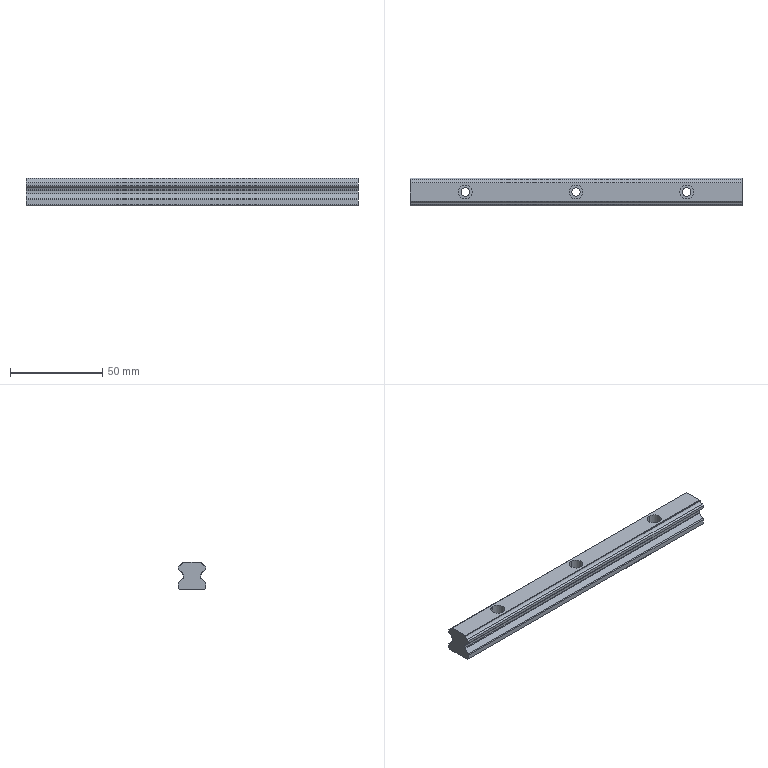Component | SolidWorks | LinearGuideHIWINHG15R150-C-1 | 1 solid | 51 faces | box 180 x 15 x 15 mm | volume 33171 mm3 | cylinder 26 | plane 25 | commonest cylinder face diameters 0.8 x8 4.5 x6 7.5 x6 3.24 x4 2 x2